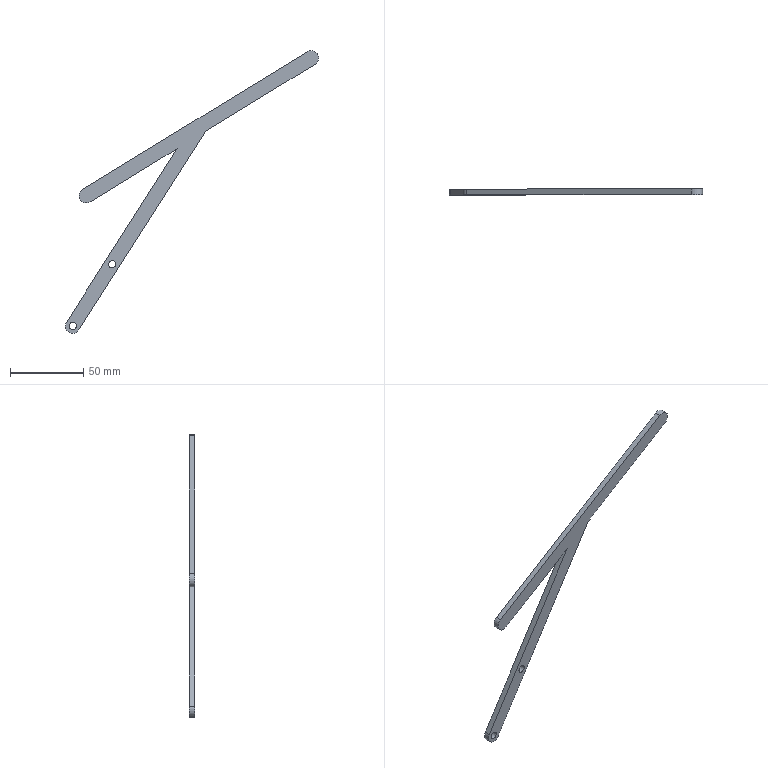Component | NX | WIPER | 1 solid | 12 faces | box 172.82 x 4 x 192.92 mm | volume 13538 mm3 | plane 7 | cylinder 5 | commonest cylinder face diameters 10 x3 5 x2
STEP:
#1=CARTESIAN_POINT('',(0.,0.,0.));
#2=DIRECTION('',(0.,0.,1.));
#3=DIRECTION('',(1.,0.,0.));
#4=AXIS2_PLACEMENT_3D('',#1,#2,#3);
#5=CARTESIAN_POINT('',(454.373,501.538,51.068));
#6=VERTEX_POINT('',#5);
#7=CARTESIAN_POINT('',(459.594,501.538,42.539));
#8=VERTEX_POINT('',#7);
#9=CARTESIAN_POINT('',(456.984,501.538,46.803));
#10=DIRECTION('',(0.,-1.,0.));
#11=DIRECTION('',(0.8431,0.,-0.5378));
#12=AXIS2_PLACEMENT_3D('',#9,#10,#11);
#13=CIRCLE('',#12,5.);
#14=CARTESIAN_POINT('',(456.984,497.538,46.803));
#15=DIRECTION('',(0.,1.,0.));
#16=DIRECTION('',(0.5378,0.,0.8431));
#17=AXIS2_PLACEMENT_3D('',#14,#15,#16);
#18=CYLINDRICAL_SURFACE('',#17,5.);
#19=CARTESIAN_POINT('',(7.854,4.));
#20=DIRECTION('',(-1.,0.));
#21=VECTOR('',#20,1.);
#22=LINE('',#19,#21);
#23=(GEOMETRIC_REPRESENTATION_CONTEXT(2)PARAMETRIC_REPRESENTATION_CONTEXT()REPRESENTATION_CONTEXT('',''));
#24=DEFINITIONAL_REPRESENTATION('',(#22),#23);
#25=PCURVE('',#18,#24);
#26=CARTESIAN_POINT('',(456.984,501.538,46.803));
#27=DIRECTION('',(0.,-1.,0.));
#28=DIRECTION('',(-0.5378,0.,-0.8431));
#29=AXIS2_PLACEMENT_3D('',#26,#27,#28);
#30=PLANE('',#29);
#31=CARTESIAN_POINT('',(0.,0.));
#32=DIRECTION('',(0.,1.));
#33=AXIS2_PLACEMENT_2D('',#31,#32);
#34=CIRCLE('',#33,5.);
#35=(GEOMETRIC_REPRESENTATION_CONTEXT(2)PARAMETRIC_REPRESENTATION_CONTEXT()REPRESENTATION_CONTEXT('',''));
#36=DEFINITIONAL_REPRESENTATION('',(#34),#35);
#37=PCURVE('',#30,#36);
#38=SURFACE_CURVE('',#13,(#25,#37),.PCURVE_S1.);
#39=EDGE_CURVE('',#6,#8,#38,.T.);
#40=ORIENTED_EDGE('',*,*,#39,.T.);
#41=CARTESIAN_POINT('',(459.594,497.538,42.539));
#42=VERTEX_POINT('',#41);
#43=CARTESIAN_POINT('',(459.594,497.538,42.539));
#44=DIRECTION('',(0.,1.,0.));
#45=VECTOR('',#44,1.);
#46=LINE('',#43,#45);
#47=CARTESIAN_POINT('',(2.025,0.));
#48=DIRECTION('',(0.,1.));
#49=VECTOR('',#48,1.);
#50=LINE('',#47,#49);
#51=(GEOMETRIC_REPRESENTATION_CONTEXT(2)PARAMETRIC_REPRESENTATION_CONTEXT()REPRESENTATION_CONTEXT('',''));
#52=DEFINITIONAL_REPRESENTATION('',(#50),#51);
#53=PCURVE('',#18,#52);
#54=CARTESIAN_POINT('',(459.594,497.538,42.539));
#55=DIRECTION('',(-0.522,0.,0.8529));
#56=DIRECTION('',(-0.8529,0.,-0.522));
#57=AXIS2_PLACEMENT_3D('',#54,#55,#56);
#58=PLANE('',#57);
#59=CARTESIAN_POINT('',(0.,0.));
#60=DIRECTION('',(0.,-1.));
#61=VECTOR('',#60,1.);
#62=LINE('',#59,#61);
#63=(GEOMETRIC_REPRESENTATION_CONTEXT(2)PARAMETRIC_REPRESENTATION_CONTEXT()REPRESENTATION_CONTEXT('',''));
#64=DEFINITIONAL_REPRESENTATION('',(#62),#63);
#65=PCURVE('',#58,#64);
#66=SURFACE_CURVE('',#46,(#53,#65),.PCURVE_S1.);
#67=EDGE_CURVE('',#42,#8,#66,.T.);
#68=ORIENTED_EDGE('',*,*,#67,.F.);
#69=CARTESIAN_POINT('',(454.373,497.538,51.068));
#70=VERTEX_POINT('',#69);
#71=CARTESIAN_POINT('',(456.984,497.538,46.803));
#72=DIRECTION('',(0.,-1.,0.));
#73=DIRECTION('',(0.8431,0.,-0.5378));
#74=AXIS2_PLACEMENT_3D('',#71,#72,#73);
#75=CIRCLE('',#74,5.);
#76=CARTESIAN_POINT('',(7.854,0.));
#77=DIRECTION('',(-1.,0.));
#78=VECTOR('',#77,1.);
#79=LINE('',#76,#78);
#80=(GEOMETRIC_REPRESENTATION_CONTEXT(2)PARAMETRIC_REPRESENTATION_CONTEXT()REPRESENTATION_CONTEXT('',''));
#81=DEFINITIONAL_REPRESENTATION('',(#79),#80);
#82=PCURVE('',#18,#81);
#83=CARTESIAN_POINT('',(456.984,497.538,46.803));
#84=DIRECTION('',(0.,-1.,0.));
#85=DIRECTION('',(-0.5378,0.,-0.8431));
#86=AXIS2_PLACEMENT_3D('',#83,#84,#85);
#87=PLANE('',#86);
#88=CARTESIAN_POINT('',(0.,0.));
#89=DIRECTION('',(0.,1.));
#90=AXIS2_PLACEMENT_2D('',#88,#89);
#91=CIRCLE('',#90,5.);
#92=(GEOMETRIC_REPRESENTATION_CONTEXT(2)PARAMETRIC_REPRESENTATION_CONTEXT()REPRESENTATION_CONTEXT('',''));
#93=DEFINITIONAL_REPRESENTATION('',(#91),#92);
#94=PCURVE('',#87,#93);
#95=SURFACE_CURVE('',#75,(#82,#94),.PCURVE_S1.);
#96=EDGE_CURVE('',#70,#42,#95,.T.);
#97=ORIENTED_EDGE('',*,*,#96,.F.);
#98=CARTESIAN_POINT('',(454.373,497.538,51.068));
#99=DIRECTION('',(0.,1.,0.));
#100=VECTOR('',#99,1.);
#101=LINE('',#98,#100);
#102=CARTESIAN_POINT('',(5.166,0.));
#103=DIRECTION('',(0.,1.));
#104=VECTOR('',#103,1.);
#105=LINE('',#102,#104);
#106=(GEOMETRIC_REPRESENTATION_CONTEXT(2)PARAMETRIC_REPRESENTATION_CONTEXT()REPRESENTATION_CONTEXT('',''));
#107=DEFINITIONAL_REPRESENTATION('',(#105),#106);
#108=PCURVE('',#18,#107);
#109=CARTESIAN_POINT('',(607.901,497.538,145.033));
#110=DIRECTION('',(0.522,0.,-0.8529));
#111=DIRECTION('',(0.8529,0.,0.522));
#112=AXIS2_PLACEMENT_3D('',#109,#110,#111);
#113=PLANE('',#112);
#114=CARTESIAN_POINT('',(-180.,0.));
#115=DIRECTION('',(0.,-1.));
#116=VECTOR('',#115,1.);
#117=LINE('',#114,#116);
#118=(GEOMETRIC_REPRESENTATION_CONTEXT(2)PARAMETRIC_REPRESENTATION_CONTEXT()REPRESENTATION_CONTEXT('',''));
#119=DEFINITIONAL_REPRESENTATION('',(#117),#118);
#120=PCURVE('',#113,#119);
#121=SURFACE_CURVE('',#101,(#108,#120),.PCURVE_S1.);
#122=EDGE_CURVE('',#70,#6,#121,.T.);
#123=ORIENTED_EDGE('',*,*,#122,.T.);
#124=EDGE_LOOP('',(#40,#68,#97,#123));
#125=FACE_BOUND('',#124,.T.);
#126=ADVANCED_FACE('',(#125),#18,.T.);
#127=CARTESIAN_POINT('',(518.949,501.538,78.866));
#128=VERTEX_POINT('',#127);
#129=CARTESIAN_POINT('',(459.594,501.538,42.539));
#130=DIRECTION('',(0.8529,0.,0.522));
#131=VECTOR('',#130,1.);
#132=LINE('',#129,#131);
#133=CARTESIAN_POINT('',(0.,-4.));
#134=DIRECTION('',(-1.,0.));
#135=VECTOR('',#134,1.);
#136=LINE('',#133,#135);
#137=(GEOMETRIC_REPRESENTATION_CONTEXT(2)PARAMETRIC_REPRESENTATION_CONTEXT()REPRESENTATION_CONTEXT('',''));
#138=DEFINITIONAL_REPRESENTATION('',(#136),#137);
#139=PCURVE('',#58,#138);
#140=CARTESIAN_POINT('',(2.192,4.494));
#141=DIRECTION('',(-0.8988,0.4384));
#142=VECTOR('',#141,1.);
#143=LINE('',#140,#142);
#144=(GEOMETRIC_REPRESENTATION_CONTEXT(2)PARAMETRIC_REPRESENTATION_CONTEXT()REPRESENTATION_CONTEXT('',''));
#145=DEFINITIONAL_REPRESENTATION('',(#143),#144);
#146=PCURVE('',#30,#145);
#147=SURFACE_CURVE('',#132,(#139,#146),.PCURVE_S1.);
#148=EDGE_CURVE('',#8,#128,#147,.T.);
#149=ORIENTED_EDGE('',*,*,#148,.T.);
#150=CARTESIAN_POINT('',(518.949,497.538,78.866));
#151=VERTEX_POINT('',#150);
#152=CARTESIAN_POINT('',(518.949,497.538,78.866));
#153=DIRECTION('',(0.,1.,0.));
#154=VECTOR('',#153,1.);
#155=LINE('',#152,#154);
#156=CARTESIAN_POINT('',(-69.59,0.));
#157=DIRECTION('',(0.,-1.));
#158=VECTOR('',#157,1.);
#159=LINE('',#156,#158);
#160=(GEOMETRIC_REPRESENTATION_CONTEXT(2)PARAMETRIC_REPRESENTATION_CONTEXT()REPRESENTATION_CONTEXT('',''));
#161=DEFINITIONAL_REPRESENTATION('',(#159),#160);
#162=PCURVE('',#58,#161);
#163=CARTESIAN_POINT('',(518.949,497.538,78.866));
#164=DIRECTION('',(0.8431,0.,-0.5378));
#165=DIRECTION('',(0.5378,0.,0.8431));
#166=AXIS2_PLACEMENT_3D('',#163,#164,#165);
#167=PLANE('',#166);
#168=CARTESIAN_POINT('',(0.,0.));
#169=DIRECTION('',(0.,-1.));
#170=VECTOR('',#169,1.);
#171=LINE('',#168,#170);
#172=(GEOMETRIC_REPRESENTATION_CONTEXT(2)PARAMETRIC_REPRESENTATION_CONTEXT()REPRESENTATION_CONTEXT('',''));
#173=DEFINITIONAL_REPRESENTATION('',(#171),#172);
#174=PCURVE('',#167,#173);
#175=SURFACE_CURVE('',#155,(#162,#174),.PCURVE_S1.);
#176=EDGE_CURVE('',#151,#128,#175,.T.);
#177=ORIENTED_EDGE('',*,*,#176,.F.);
#178=CARTESIAN_POINT('',(459.594,497.538,42.539));
#179=DIRECTION('',(0.8529,0.,0.522));
#180=VECTOR('',#179,1.);
#181=LINE('',#178,#180);
#182=CARTESIAN_POINT('',(0.,0.));
#183=DIRECTION('',(-1.,0.));
#184=VECTOR('',#183,1.);
#185=LINE('',#182,#184);
#186=(GEOMETRIC_REPRESENTATION_CONTEXT(2)PARAMETRIC_REPRESENTATION_CONTEXT()REPRESENTATION_CONTEXT('',''));
#187=DEFINITIONAL_REPRESENTATION('',(#185),#186);
#188=PCURVE('',#58,#187);
#189=CARTESIAN_POINT('',(2.192,4.494));
#190=DIRECTION('',(-0.8988,0.4384));
#191=VECTOR('',#190,1.);
#192=LINE('',#189,#191);
#193=(GEOMETRIC_REPRESENTATION_CONTEXT(2)PARAMETRIC_REPRESENTATION_CONTEXT()REPRESENTATION_CONTEXT('',''));
#194=DEFINITIONAL_REPRESENTATION('',(#192),#193);
#195=PCURVE('',#87,#194);
#196=SURFACE_CURVE('',#181,(#188,#195),.PCURVE_S1.);
#197=EDGE_CURVE('',#42,#151,#196,.T.);
#198=ORIENTED_EDGE('',*,*,#197,.F.);
#199=ORIENTED_EDGE('',*,*,#67,.T.);
#200=EDGE_LOOP('',(#149,#177,#198,#199));
#201=FACE_BOUND('',#200,.T.);
#202=ADVANCED_FACE('',(#201),#58,.F.);
#203=CARTESIAN_POINT('',(443.471,501.538,-39.466));
#204=VERTEX_POINT('',#203);
#205=CARTESIAN_POINT('',(518.949,501.538,78.866));
#206=DIRECTION('',(-0.5378,0.,-0.8431));
#207=VECTOR('',#206,1.);
#208=LINE('',#205,#207);
#209=CARTESIAN_POINT('',(0.,-4.));
#210=DIRECTION('',(-1.,0.));
#211=VECTOR('',#210,1.);
#212=LINE('',#209,#211);
#213=(GEOMETRIC_REPRESENTATION_CONTEXT(2)PARAMETRIC_REPRESENTATION_CONTEXT()REPRESENTATION_CONTEXT('',''));
#214=DEFINITIONAL_REPRESENTATION('',(#212),#213);
#215=PCURVE('',#167,#214);
#216=CARTESIAN_POINT('',(-60.355,35.));
#217=DIRECTION('',(1.,0.));
#218=VECTOR('',#217,1.);
#219=LINE('',#216,#218);
#220=(GEOMETRIC_REPRESENTATION_CONTEXT(2)PARAMETRIC_REPRESENTATION_CONTEXT()REPRESENTATION_CONTEXT('',''));
#221=DEFINITIONAL_REPRESENTATION('',(#219),#220);
#222=PCURVE('',#30,#221);
#223=SURFACE_CURVE('',#208,(#215,#222),.PCURVE_S1.);
#224=EDGE_CURVE('',#128,#204,#223,.T.);
#225=ORIENTED_EDGE('',*,*,#224,.T.);
#226=CARTESIAN_POINT('',(443.471,497.538,-39.466));
#227=VERTEX_POINT('',#226);
#228=CARTESIAN_POINT('',(443.471,497.538,-39.466));
#229=DIRECTION('',(0.,1.,0.));
#230=VECTOR('',#229,1.);
#231=LINE('',#228,#230);
#232=CARTESIAN_POINT('',(-140.355,0.));
#233=DIRECTION('',(0.,-1.));
#234=VECTOR('',#233,1.);
#235=LINE('',#232,#234);
#236=(GEOMETRIC_REPRESENTATION_CONTEXT(2)PARAMETRIC_REPRESENTATION_CONTEXT()REPRESENTATION_CONTEXT('',''));
#237=DEFINITIONAL_REPRESENTATION('',(#235),#236);
#238=PCURVE('',#167,#237);
#239=CARTESIAN_POINT('',(447.686,497.538,-42.155));
#240=DIRECTION('',(0.,1.,0.));
#241=DIRECTION('',(0.5378,0.,0.8431));
#242=AXIS2_PLACEMENT_3D('',#239,#240,#241);
#243=CYLINDRICAL_SURFACE('',#242,5.);
#244=CARTESIAN_POINT('',(4.712,0.));
#245=DIRECTION('',(0.,1.));
#246=VECTOR('',#245,1.);
#247=LINE('',#244,#246);
#248=(GEOMETRIC_REPRESENTATION_CONTEXT(2)PARAMETRIC_REPRESENTATION_CONTEXT()REPRESENTATION_CONTEXT('',''));
#249=DEFINITIONAL_REPRESENTATION('',(#247),#248);
#250=PCURVE('',#243,#249);
#251=SURFACE_CURVE('',#231,(#238,#250),.PCURVE_S1.);
#252=EDGE_CURVE('',#227,#204,#251,.T.);
#253=ORIENTED_EDGE('',*,*,#252,.F.);
#254=CARTESIAN_POINT('',(518.949,497.538,78.866));
#255=DIRECTION('',(-0.5378,0.,-0.8431));
#256=VECTOR('',#255,1.);
#257=LINE('',#254,#256);
#258=CARTESIAN_POINT('',(0.,0.));
#259=DIRECTION('',(-1.,0.));
#260=VECTOR('',#259,1.);
#261=LINE('',#258,#260);
#262=(GEOMETRIC_REPRESENTATION_CONTEXT(2)PARAMETRIC_REPRESENTATION_CONTEXT()REPRESENTATION_CONTEXT('',''));
#263=DEFINITIONAL_REPRESENTATION('',(#261),#262);
#264=PCURVE('',#167,#263);
#265=CARTESIAN_POINT('',(-60.355,35.));
#266=DIRECTION('',(1.,0.));
#267=VECTOR('',#266,1.);
#268=LINE('',#265,#267);
#269=(GEOMETRIC_REPRESENTATION_CONTEXT(2)PARAMETRIC_REPRESENTATION_CONTEXT()REPRESENTATION_CONTEXT('',''));
#270=DEFINITIONAL_REPRESENTATION('',(#268),#269);
#271=PCURVE('',#87,#270);
#272=SURFACE_CURVE('',#257,(#264,#271),.PCURVE_S1.);
#273=EDGE_CURVE('',#151,#227,#272,.T.);
#274=ORIENTED_EDGE('',*,*,#273,.F.);
#275=ORIENTED_EDGE('',*,*,#176,.T.);
#276=EDGE_LOOP('',(#225,#253,#274,#275));
#277=FACE_BOUND('',#276,.T.);
#278=ADVANCED_FACE('',(#277),#167,.F.);
#279=CARTESIAN_POINT('',(451.901,501.538,-44.844));
#280=VERTEX_POINT('',#279);
#281=CARTESIAN_POINT('',(447.686,501.538,-42.155));
#282=DIRECTION('',(0.,-1.,0.));
#283=DIRECTION('',(0.8431,0.,-0.5378));
#284=AXIS2_PLACEMENT_3D('',#281,#282,#283);
#285=CIRCLE('',#284,5.);
#286=CARTESIAN_POINT('',(7.854,4.));
#287=DIRECTION('',(-1.,0.));
#288=VECTOR('',#287,1.);
#289=LINE('',#286,#288);
#290=(GEOMETRIC_REPRESENTATION_CONTEXT(2)PARAMETRIC_REPRESENTATION_CONTEXT()REPRESENTATION_CONTEXT('',''));
#291=DEFINITIONAL_REPRESENTATION('',(#289),#290);
#292=PCURVE('',#243,#291);
#293=CARTESIAN_POINT('',(80.,40.));
#294=DIRECTION('',(0.,1.));
#295=AXIS2_PLACEMENT_2D('',#293,#294);
#296=CIRCLE('',#295,5.);
#297=(GEOMETRIC_REPRESENTATION_CONTEXT(2)PARAMETRIC_REPRESENTATION_CONTEXT()REPRESENTATION_CONTEXT('',''));
#298=DEFINITIONAL_REPRESENTATION('',(#296),#297);
#299=PCURVE('',#30,#298);
#300=SURFACE_CURVE('',#285,(#292,#299),.PCURVE_S1.);
#301=EDGE_CURVE('',#204,#280,#300,.T.);
#302=ORIENTED_EDGE('',*,*,#301,.T.);
#303=CARTESIAN_POINT('',(451.901,497.538,-44.844));
#304=VERTEX_POINT('',#303);
#305=CARTESIAN_POINT('',(451.901,497.538,-44.844));
#306=DIRECTION('',(0.,1.,0.));
#307=VECTOR('',#306,1.);
#308=LINE('',#305,#307);
#309=CARTESIAN_POINT('',(1.571,0.));
#310=DIRECTION('',(0.,1.));
#311=VECTOR('',#310,1.);
#312=LINE('',#309,#311);
#313=(GEOMETRIC_REPRESENTATION_CONTEXT(2)PARAMETRIC_REPRESENTATION_CONTEXT()REPRESENTATION_CONTEXT('',''));
#314=DEFINITIONAL_REPRESENTATION('',(#312),#313);
#315=PCURVE('',#243,#314);
#316=CARTESIAN_POINT('',(451.901,497.538,-44.844));
#317=DIRECTION('',(-0.8431,0.,0.5378));
#318=DIRECTION('',(-0.5378,0.,-0.8431));
#319=AXIS2_PLACEMENT_3D('',#316,#317,#318);
#320=PLANE('',#319);
#321=CARTESIAN_POINT('',(0.,0.));
#322=DIRECTION('',(0.,-1.));
#323=VECTOR('',#322,1.);
#324=LINE('',#321,#323);
#325=(GEOMETRIC_REPRESENTATION_CONTEXT(2)PARAMETRIC_REPRESENTATION_CONTEXT()REPRESENTATION_CONTEXT('',''));
#326=DEFINITIONAL_REPRESENTATION('',(#324),#325);
#327=PCURVE('',#320,#326);
#328=SURFACE_CURVE('',#308,(#315,#327),.PCURVE_S1.);
#329=EDGE_CURVE('',#304,#280,#328,.T.);
#330=ORIENTED_EDGE('',*,*,#329,.F.);
#331=CARTESIAN_POINT('',(447.686,497.538,-42.155));
#332=DIRECTION('',(0.,-1.,0.));
#333=DIRECTION('',(0.8431,0.,-0.5378));
#334=AXIS2_PLACEMENT_3D('',#331,#332,#333);
#335=CIRCLE('',#334,5.);
#336=CARTESIAN_POINT('',(7.854,0.));
#337=DIRECTION('',(-1.,0.));
#338=VECTOR('',#337,1.);
#339=LINE('',#336,#338);
#340=(GEOMETRIC_REPRESENTATION_CONTEXT(2)PARAMETRIC_REPRESENTATION_CONTEXT()REPRESENTATION_CONTEXT('',''));
#341=DEFINITIONAL_REPRESENTATION('',(#339),#340);
#342=PCURVE('',#243,#341);
#343=CARTESIAN_POINT('',(80.,40.));
#344=DIRECTION('',(0.,1.));
#345=AXIS2_PLACEMENT_2D('',#343,#344);
#346=CIRCLE('',#345,5.);
#347=(GEOMETRIC_REPRESENTATION_CONTEXT(2)PARAMETRIC_REPRESENTATION_CONTEXT()REPRESENTATION_CONTEXT('',''));
#348=DEFINITIONAL_REPRESENTATION('',(#346),#347);
#349=PCURVE('',#87,#348);
#350=SURFACE_CURVE('',#335,(#342,#349),.PCURVE_S1.);
#351=EDGE_CURVE('',#227,#304,#350,.T.);
#352=ORIENTED_EDGE('',*,*,#351,.F.);
#353=ORIENTED_EDGE('',*,*,#252,.T.);
#354=EDGE_LOOP('',(#302,#330,#352,#353));
#355=FACE_BOUND('',#354,.T.);
#356=ADVANCED_FACE('',(#355),#243,.T.);
#357=CARTESIAN_POINT('',(538.405,501.538,90.775));
#358=VERTEX_POINT('',#357);
#359=CARTESIAN_POINT('',(451.901,501.538,-44.844));
#360=DIRECTION('',(0.5378,0.,0.8431));
#361=VECTOR('',#360,1.);
#362=LINE('',#359,#361);
#363=CARTESIAN_POINT('',(0.,-4.));
#364=DIRECTION('',(-1.,0.));
#365=VECTOR('',#364,1.);
#366=LINE('',#363,#365);
#367=(GEOMETRIC_REPRESENTATION_CONTEXT(2)PARAMETRIC_REPRESENTATION_CONTEXT()REPRESENTATION_CONTEXT('',''));
#368=DEFINITIONAL_REPRESENTATION('',(#366),#367);
#369=PCURVE('',#320,#368);
#370=CARTESIAN_POINT('',(80.,45.));
#371=DIRECTION('',(-1.,0.));
#372=VECTOR('',#371,1.);
#373=LINE('',#370,#372);
#374=(GEOMETRIC_REPRESENTATION_CONTEXT(2)PARAMETRIC_REPRESENTATION_CONTEXT()REPRESENTATION_CONTEXT('',''));
#375=DEFINITIONAL_REPRESENTATION('',(#373),#374);
#376=PCURVE('',#30,#375);
#377=SURFACE_CURVE('',#362,(#369,#376),.PCURVE_S1.);
#378=EDGE_CURVE('',#280,#358,#377,.T.);
#379=ORIENTED_EDGE('',*,*,#378,.T.);
#380=CARTESIAN_POINT('',(538.405,497.538,90.775));
#381=VERTEX_POINT('',#380);
#382=CARTESIAN_POINT('',(538.405,497.538,90.775));
#383=DIRECTION('',(0.,1.,0.));
#384=VECTOR('',#383,1.);
#385=LINE('',#382,#384);
#386=CARTESIAN_POINT('',(-160.858,0.));
#387=DIRECTION('',(0.,-1.));
#388=VECTOR('',#387,1.);
#389=LINE('',#386,#388);
#390=(GEOMETRIC_REPRESENTATION_CONTEXT(2)PARAMETRIC_REPRESENTATION_CONTEXT()REPRESENTATION_CONTEXT('',''));
#391=DEFINITIONAL_REPRESENTATION('',(#389),#390);
#392=PCURVE('',#320,#391);
#393=CARTESIAN_POINT('',(538.405,497.538,90.775));
#394=DIRECTION('',(-0.522,0.,0.8529));
#395=DIRECTION('',(-0.8529,0.,-0.522));
#396=AXIS2_PLACEMENT_3D('',#393,#394,#395);
#397=PLANE('',#396);
#398=CARTESIAN_POINT('',(0.,0.));
#399=DIRECTION('',(0.,-1.));
#400=VECTOR('',#399,1.);
#401=LINE('',#398,#400);
#402=(GEOMETRIC_REPRESENTATION_CONTEXT(2)PARAMETRIC_REPRESENTATION_CONTEXT()REPRESENTATION_CONTEXT('',''));
#403=DEFINITIONAL_REPRESENTATION('',(#401),#402);
#404=PCURVE('',#397,#403);
#405=SURFACE_CURVE('',#385,(#392,#404),.PCURVE_S1.);
#406=EDGE_CURVE('',#381,#358,#405,.T.);
#407=ORIENTED_EDGE('',*,*,#406,.F.);
#408=CARTESIAN_POINT('',(451.901,497.538,-44.844));
#409=DIRECTION('',(0.5378,0.,0.8431));
#410=VECTOR('',#409,1.);
#411=LINE('',#408,#410);
#412=CARTESIAN_POINT('',(0.,0.));
#413=DIRECTION('',(-1.,0.));
#414=VECTOR('',#413,1.);
#415=LINE('',#412,#414);
#416=(GEOMETRIC_REPRESENTATION_CONTEXT(2)PARAMETRIC_REPRESENTATION_CONTEXT()REPRESENTATION_CONTEXT('',''));
#417=DEFINITIONAL_REPRESENTATION('',(#415),#416);
#418=PCURVE('',#320,#417);
#419=CARTESIAN_POINT('',(80.,45.));
#420=DIRECTION('',(-1.,0.));
#421=VECTOR('',#420,1.);
#422=LINE('',#419,#421);
#423=(GEOMETRIC_REPRESENTATION_CONTEXT(2)PARAMETRIC_REPRESENTATION_CONTEXT()REPRESENTATION_CONTEXT('',''));
#424=DEFINITIONAL_REPRESENTATION('',(#422),#423);
#425=PCURVE('',#87,#424);
#426=SURFACE_CURVE('',#411,(#418,#425),.PCURVE_S1.);
#427=EDGE_CURVE('',#304,#381,#426,.T.);
#428=ORIENTED_EDGE('',*,*,#427,.F.);
#429=ORIENTED_EDGE('',*,*,#329,.T.);
#430=EDGE_LOOP('',(#379,#407,#428,#429));
#431=FACE_BOUND('',#430,.T.);
#432=ADVANCED_FACE('',(#431),#320,.F.);
#433=CARTESIAN_POINT('',(613.121,501.538,136.504));
#434=VERTEX_POINT('',#433);
#435=CARTESIAN_POINT('',(538.405,501.538,90.775));
#436=DIRECTION('',(0.8529,0.,0.522));
#437=VECTOR('',#436,1.);
#438=LINE('',#435,#437);
#439=CARTESIAN_POINT('',(0.,-4.));
#440=DIRECTION('',(-1.,0.));
#441=VECTOR('',#440,1.);
#442=LINE('',#439,#441);
#443=(GEOMETRIC_REPRESENTATION_CONTEXT(2)PARAMETRIC_REPRESENTATION_CONTEXT()REPRESENTATION_CONTEXT('',''));
#444=DEFINITIONAL_REPRESENTATION('',(#442),#443);
#445=PCURVE('',#397,#444);
#446=CARTESIAN_POINT('',(-80.858,45.));
#447=DIRECTION('',(-0.8988,0.4384));
#448=VECTOR('',#447,1.);
#449=LINE('',#446,#448);
#450=(GEOMETRIC_REPRESENTATION_CONTEXT(2)PARAMETRIC_REPRESENTATION_CONTEXT()REPRESENTATION_CONTEXT('',''));
#451=DEFINITIONAL_REPRESENTATION('',(#449),#450);
#452=PCURVE('',#30,#451);
#453=SURFACE_CURVE('',#438,(#445,#452),.PCURVE_S1.);
#454=EDGE_CURVE('',#358,#434,#453,.T.);
#455=ORIENTED_EDGE('',*,*,#454,.T.);
#456=CARTESIAN_POINT('',(613.121,497.538,136.504));
#457=VERTEX_POINT('',#456);
#458=CARTESIAN_POINT('',(613.121,497.538,136.504));
#459=DIRECTION('',(0.,1.,0.));
#460=VECTOR('',#459,1.);
#461=LINE('',#458,#460);
#462=CARTESIAN_POINT('',(-87.599,0.));
#463=DIRECTION('',(0.,-1.));
#464=VECTOR('',#463,1.);
#465=LINE('',#462,#464);
#466=(GEOMETRIC_REPRESENTATION_CONTEXT(2)PARAMETRIC_REPRESENTATION_CONTEXT()REPRESENTATION_CONTEXT('',''));
#467=DEFINITIONAL_REPRESENTATION('',(#465),#466);
#468=PCURVE('',#397,#467);
#469=CARTESIAN_POINT('',(610.511,497.538,140.768));
#470=DIRECTION('',(0.,1.,0.));
#471=DIRECTION('',(0.5378,0.,0.8431));
#472=AXIS2_PLACEMENT_3D('',#469,#470,#471);
#473=CYLINDRICAL_SURFACE('',#472,5.);
#474=CARTESIAN_POINT('',(2.025,0.));
#475=DIRECTION('',(0.,1.));
#476=VECTOR('',#475,1.);
#477=LINE('',#474,#476);
#478=(GEOMETRIC_REPRESENTATION_CONTEXT(2)PARAMETRIC_REPRESENTATION_CONTEXT()REPRESENTATION_CONTEXT('',''));
#479=DEFINITIONAL_REPRESENTATION('',(#477),#478);
#480=PCURVE('',#473,#479);
#481=SURFACE_CURVE('',#461,(#468,#480),.PCURVE_S1.);
#482=EDGE_CURVE('',#457,#434,#481,.T.);
#483=ORIENTED_EDGE('',*,*,#482,.F.);
#484=CARTESIAN_POINT('',(538.405,497.538,90.775));
#485=DIRECTION('',(0.8529,0.,0.522));
#486=VECTOR('',#485,1.);
#487=LINE('',#484,#486);
#488=CARTESIAN_POINT('',(0.,0.));
#489=DIRECTION('',(-1.,0.));
#490=VECTOR('',#489,1.);
#491=LINE('',#488,#490);
#492=(GEOMETRIC_REPRESENTATION_CONTEXT(2)PARAMETRIC_REPRESENTATION_CONTEXT()REPRESENTATION_CONTEXT('',''));
#493=DEFINITIONAL_REPRESENTATION('',(#491),#492);
#494=PCURVE('',#397,#493);
#495=CARTESIAN_POINT('',(-80.858,45.));
#496=DIRECTION('',(-0.8988,0.4384));
#497=VECTOR('',#496,1.);
#498=LINE('',#495,#497);
#499=(GEOMETRIC_REPRESENTATION_CONTEXT(2)PARAMETRIC_REPRESENTATION_CONTEXT()REPRESENTATION_CONTEXT('',''));
#500=DEFINITIONAL_REPRESENTATION('',(#498),#499);
#501=PCURVE('',#87,#500);
#502=SURFACE_CURVE('',#487,(#494,#501),.PCURVE_S1.);
#503=EDGE_CURVE('',#381,#457,#502,.T.);
#504=ORIENTED_EDGE('',*,*,#503,.F.);
#505=ORIENTED_EDGE('',*,*,#406,.T.);
#506=EDGE_LOOP('',(#455,#483,#504,#505));
#507=FACE_BOUND('',#506,.T.);
#508=ADVANCED_FACE('',(#507),#397,.F.);
#509=CARTESIAN_POINT('',(607.901,501.538,145.033));
#510=VERTEX_POINT('',#509);
#511=CARTESIAN_POINT('',(610.511,501.538,140.768));
#512=DIRECTION('',(0.,-1.,0.));
#513=DIRECTION('',(0.8431,0.,-0.5378));
#514=AXIS2_PLACEMENT_3D('',#511,#512,#513);
#515=CIRCLE('',#514,5.);
#516=CARTESIAN_POINT('',(7.854,4.));
#517=DIRECTION('',(-1.,0.));
#518=VECTOR('',#517,1.);
#519=LINE('',#516,#518);
#520=(GEOMETRIC_REPRESENTATION_CONTEXT(2)PARAMETRIC_REPRESENTATION_CONTEXT()REPRESENTATION_CONTEXT('',''));
#521=DEFINITIONAL_REPRESENTATION('',(#519),#520);
#522=PCURVE('',#473,#521);
#523=CARTESIAN_POINT('',(-161.783,78.907));
#524=DIRECTION('',(-0.,1.));
#525=AXIS2_PLACEMENT_2D('',#523,#524);
#526=CIRCLE('',#525,5.);
#527=(GEOMETRIC_REPRESENTATION_CONTEXT(2)PARAMETRIC_REPRESENTATION_CONTEXT()REPRESENTATION_CONTEXT('',''));
#528=DEFINITIONAL_REPRESENTATION('',(#526),#527);
#529=PCURVE('',#30,#528);
#530=SURFACE_CURVE('',#515,(#522,#529),.PCURVE_S1.);
#531=EDGE_CURVE('',#434,#510,#530,.T.);
#532=ORIENTED_EDGE('',*,*,#531,.T.);
#533=CARTESIAN_POINT('',(607.901,497.538,145.033));
#534=VERTEX_POINT('',#533);
#535=CARTESIAN_POINT('',(607.901,497.538,145.033));
#536=DIRECTION('',(0.,1.,0.));
#537=VECTOR('',#536,1.);
#538=LINE('',#535,#537);
#539=CARTESIAN_POINT('',(-1.117,0.));
#540=DIRECTION('',(0.,1.));
#541=VECTOR('',#540,1.);
#542=LINE('',#539,#541);
#543=(GEOMETRIC_REPRESENTATION_CONTEXT(2)PARAMETRIC_REPRESENTATION_CONTEXT()REPRESENTATION_CONTEXT('',''));
#544=DEFINITIONAL_REPRESENTATION('',(#542),#543);
#545=PCURVE('',#473,#544);
#546=CARTESIAN_POINT('',(0.,0.));
#547=DIRECTION('',(0.,-1.));
#548=VECTOR('',#547,1.);
#549=LINE('',#546,#548);
#550=(GEOMETRIC_REPRESENTATION_CONTEXT(2)PARAMETRIC_REPRESENTATION_CONTEXT()REPRESENTATION_CONTEXT('',''));
#551=DEFINITIONAL_REPRESENTATION('',(#549),#550);
#552=PCURVE('',#113,#551);
#553=SURFACE_CURVE('',#538,(#545,#552),.PCURVE_S1.);
#554=EDGE_CURVE('',#534,#510,#553,.T.);
#555=ORIENTED_EDGE('',*,*,#554,.F.);
#556=CARTESIAN_POINT('',(610.511,497.538,140.768));
#557=DIRECTION('',(0.,-1.,0.));
#558=DIRECTION('',(0.8431,0.,-0.5378));
#559=AXIS2_PLACEMENT_3D('',#556,#557,#558);
#560=CIRCLE('',#559,5.);
#561=CARTESIAN_POINT('',(7.854,0.));
#562=DIRECTION('',(-1.,0.));
#563=VECTOR('',#562,1.);
#564=LINE('',#561,#563);
#565=(GEOMETRIC_REPRESENTATION_CONTEXT(2)PARAMETRIC_REPRESENTATION_CONTEXT()REPRESENTATION_CONTEXT('',''));
#566=DEFINITIONAL_REPRESENTATION('',(#564),#565);
#567=PCURVE('',#473,#566);
#568=CARTESIAN_POINT('',(-161.783,78.907));
#569=DIRECTION('',(-0.,1.));
#570=AXIS2_PLACEMENT_2D('',#568,#569);
#571=CIRCLE('',#570,5.);
#572=(GEOMETRIC_REPRESENTATION_CONTEXT(2)PARAMETRIC_REPRESENTATION_CONTEXT()REPRESENTATION_CONTEXT('',''));
#573=DEFINITIONAL_REPRESENTATION('',(#571),#572);
#574=PCURVE('',#87,#573);
#575=SURFACE_CURVE('',#560,(#567,#574),.PCURVE_S1.);
#576=EDGE_CURVE('',#457,#534,#575,.T.);
#577=ORIENTED_EDGE('',*,*,#576,.F.);
#578=ORIENTED_EDGE('',*,*,#482,.T.);
#579=EDGE_LOOP('',(#532,#555,#577,#578));
#580=FACE_BOUND('',#579,.T.);
#581=ADVANCED_FACE('',(#580),#473,.T.);
#582=CARTESIAN_POINT('',(449.794,497.538,-43.499));
#583=VERTEX_POINT('',#582);
#584=CARTESIAN_POINT('',(447.686,497.538,-42.155));
#585=DIRECTION('',(0.,-1.,0.));
#586=DIRECTION('',(0.8431,0.,-0.5378));
#587=AXIS2_PLACEMENT_3D('',#584,#585,#586);
#588=CIRCLE('',#587,2.5);
#589=CARTESIAN_POINT('',(447.686,497.538,-42.155));
#590=DIRECTION('',(0.,1.,0.));
#591=DIRECTION('',(0.5378,0.,0.8431));
#592=AXIS2_PLACEMENT_3D('',#589,#590,#591);
#593=CYLINDRICAL_SURFACE('',#592,2.5);
#594=CARTESIAN_POINT('',(7.854,0.));
#595=DIRECTION('',(-1.,0.));
#596=VECTOR('',#595,1.);
#597=LINE('',#594,#596);
#598=(GEOMETRIC_REPRESENTATION_CONTEXT(2)PARAMETRIC_REPRESENTATION_CONTEXT()REPRESENTATION_CONTEXT('',''));
#599=DEFINITIONAL_REPRESENTATION('',(#597),#598);
#600=PCURVE('',#593,#599);
#601=CARTESIAN_POINT('',(80.,40.));
#602=DIRECTION('',(0.,1.));
#603=AXIS2_PLACEMENT_2D('',#601,#602);
#604=CIRCLE('',#603,2.5);
#605=(GEOMETRIC_REPRESENTATION_CONTEXT(2)PARAMETRIC_REPRESENTATION_CONTEXT()REPRESENTATION_CONTEXT('',''));
#606=DEFINITIONAL_REPRESENTATION('',(#604),#605);
#607=PCURVE('',#87,#606);
#608=SURFACE_CURVE('',#588,(#600,#607),.PCURVE_S1.);
#609=EDGE_CURVE('',#583,#583,#608,.T.);
#610=ORIENTED_EDGE('',*,*,#609,.F.);
#611=CARTESIAN_POINT('',(449.794,501.538,-43.499));
#612=VERTEX_POINT('',#611);
#613=CARTESIAN_POINT('',(449.794,497.538,-43.499));
#614=CARTESIAN_POINT('',(449.794,501.538,-43.499));
#615=B_SPLINE_CURVE_WITH_KNOTS('',1,(#613,#614),.UNSPECIFIED.,.F.,.F.,(2,2),(0.,4.),.PIECEWISE_BEZIER_KNOTS.);
#616=CARTESIAN_POINT('',(7.854,0.));
#617=DIRECTION('',(0.,1.));
#618=VECTOR('',#617,1.);
#619=LINE('',#616,#618);
#620=(GEOMETRIC_REPRESENTATION_CONTEXT(2)PARAMETRIC_REPRESENTATION_CONTEXT()REPRESENTATION_CONTEXT('',''));
#621=DEFINITIONAL_REPRESENTATION('',(#619),#620);
#622=PCURVE('',#593,#621);
#623=CARTESIAN_POINT('',(1.571,0.));
#624=DIRECTION('',(0.,1.));
#625=VECTOR('',#624,1.);
#626=LINE('',#623,#625);
#627=(GEOMETRIC_REPRESENTATION_CONTEXT(2)PARAMETRIC_REPRESENTATION_CONTEXT()REPRESENTATION_CONTEXT('',''));
#628=DEFINITIONAL_REPRESENTATION('',(#626),#627);
#629=PCURVE('',#593,#628);
#630=SEAM_CURVE('',#615,(#622,#629),.PCURVE_S1.);
#631=EDGE_CURVE('',#583,#612,#630,.T.);
#632=ORIENTED_EDGE('',*,*,#631,.T.);
#633=CARTESIAN_POINT('',(447.686,501.538,-42.155));
#634=DIRECTION('',(0.,-1.,0.));
#635=DIRECTION('',(0.8431,0.,-0.5378));
#636=AXIS2_PLACEMENT_3D('',#633,#634,#635);
#637=CIRCLE('',#636,2.5);
#638=CARTESIAN_POINT('',(7.854,4.));
#639=DIRECTION('',(-1.,0.));
#640=VECTOR('',#639,1.);
#641=LINE('',#638,#640);
#642=(GEOMETRIC_REPRESENTATION_CONTEXT(2)PARAMETRIC_REPRESENTATION_CONTEXT()REPRESENTATION_CONTEXT('',''));
#643=DEFINITIONAL_REPRESENTATION('',(#641),#642);
#644=PCURVE('',#593,#643);
#645=CARTESIAN_POINT('',(80.,40.));
#646=DIRECTION('',(0.,1.));
#647=AXIS2_PLACEMENT_2D('',#645,#646);
#648=CIRCLE('',#647,2.5);
#649=(GEOMETRIC_REPRESENTATION_CONTEXT(2)PARAMETRIC_REPRESENTATION_CONTEXT()REPRESENTATION_CONTEXT('',''));
#650=DEFINITIONAL_REPRESENTATION('',(#648),#649);
#651=PCURVE('',#30,#650);
#652=SURFACE_CURVE('',#637,(#644,#651),.PCURVE_S1.);
#653=EDGE_CURVE('',#612,#612,#652,.T.);
#654=ORIENTED_EDGE('',*,*,#653,.T.);
#655=ORIENTED_EDGE('',*,*,#631,.F.);
#656=EDGE_LOOP('',(#610,#632,#654,#655));
#657=FACE_BOUND('',#656,.F.);
#658=ADVANCED_FACE('',(#657),#593,.F.);
#659=CARTESIAN_POINT('',(607.901,501.538,145.033));
#660=DIRECTION('',(-0.8529,0.,-0.522));
#661=VECTOR('',#660,1.);
#662=LINE('',#659,#661);
#663=CARTESIAN_POINT('',(0.,-4.));
#664=DIRECTION('',(-1.,0.));
#665=VECTOR('',#664,1.);
#666=LINE('',#663,#665);
#667=(GEOMETRIC_REPRESENTATION_CONTEXT(2)PARAMETRIC_REPRESENTATION_CONTEXT()REPRESENTATION_CONTEXT('',''));
#668=DEFINITIONAL_REPRESENTATION('',(#666),#667);
#669=PCURVE('',#113,#668);
#670=CARTESIAN_POINT('',(-163.975,74.413));
#671=DIRECTION('',(0.8988,-0.4384));
#672=VECTOR('',#671,1.);
#673=LINE('',#670,#672);
#674=(GEOMETRIC_REPRESENTATION_CONTEXT(2)PARAMETRIC_REPRESENTATION_CONTEXT()REPRESENTATION_CONTEXT('',''));
#675=DEFINITIONAL_REPRESENTATION('',(#673),#674);
#676=PCURVE('',#30,#675);
#677=SURFACE_CURVE('',#662,(#669,#676),.PCURVE_S1.);
#678=EDGE_CURVE('',#510,#6,#677,.T.);
#679=ORIENTED_EDGE('',*,*,#678,.T.);
#680=ORIENTED_EDGE('',*,*,#122,.F.);
#681=CARTESIAN_POINT('',(607.901,497.538,145.033));
#682=DIRECTION('',(-0.8529,0.,-0.522));
#683=VECTOR('',#682,1.);
#684=LINE('',#681,#683);
#685=CARTESIAN_POINT('',(0.,0.));
#686=DIRECTION('',(-1.,0.));
#687=VECTOR('',#686,1.);
#688=LINE('',#685,#687);
#689=(GEOMETRIC_REPRESENTATION_CONTEXT(2)PARAMETRIC_REPRESENTATION_CONTEXT()REPRESENTATION_CONTEXT('',''));
#690=DEFINITIONAL_REPRESENTATION('',(#688),#689);
#691=PCURVE('',#113,#690);
#692=CARTESIAN_POINT('',(-163.975,74.413));
#693=DIRECTION('',(0.8988,-0.4384));
#694=VECTOR('',#693,1.);
#695=LINE('',#692,#694);
#696=(GEOMETRIC_REPRESENTATION_CONTEXT(2)PARAMETRIC_REPRESENTATION_CONTEXT()REPRESENTATION_CONTEXT('',''));
#697=DEFINITIONAL_REPRESENTATION('',(#695),#696);
#698=PCURVE('',#87,#697);
#699=SURFACE_CURVE('',#684,(#691,#698),.PCURVE_S1.);
#700=EDGE_CURVE('',#534,#70,#699,.T.);
#701=ORIENTED_EDGE('',*,*,#700,.F.);
#702=ORIENTED_EDGE('',*,*,#554,.T.);
#703=EDGE_LOOP('',(#679,#680,#701,#702));
#704=FACE_BOUND('',#703,.T.);
#705=ADVANCED_FACE('',(#704),#113,.F.);
#706=CARTESIAN_POINT('',(476.682,497.538,-1.344));
#707=VERTEX_POINT('',#706);
#708=CARTESIAN_POINT('',(474.574,497.538,0.));
#709=DIRECTION('',(0.,-1.,0.));
#710=DIRECTION('',(0.8431,0.,-0.5378));
#711=AXIS2_PLACEMENT_3D('',#708,#709,#710);
#712=CIRCLE('',#711,2.5);
#713=CARTESIAN_POINT('',(474.574,497.538,0.));
#714=DIRECTION('',(0.,1.,0.));
#715=DIRECTION('',(0.5378,0.,0.8431));
#716=AXIS2_PLACEMENT_3D('',#713,#714,#715);
#717=CYLINDRICAL_SURFACE('',#716,2.5);
#718=CARTESIAN_POINT('',(7.854,0.));
#719=DIRECTION('',(-1.,0.));
#720=VECTOR('',#719,1.);
#721=LINE('',#718,#720);
#722=(GEOMETRIC_REPRESENTATION_CONTEXT(2)PARAMETRIC_REPRESENTATION_CONTEXT()REPRESENTATION_CONTEXT('',''));
#723=DEFINITIONAL_REPRESENTATION('',(#721),#722);
#724=PCURVE('',#717,#723);
#725=CARTESIAN_POINT('',(30.,40.));
#726=DIRECTION('',(0.,1.));
#727=AXIS2_PLACEMENT_2D('',#725,#726);
#728=CIRCLE('',#727,2.5);
#729=(GEOMETRIC_REPRESENTATION_CONTEXT(2)PARAMETRIC_REPRESENTATION_CONTEXT()REPRESENTATION_CONTEXT('',''));
#730=DEFINITIONAL_REPRESENTATION('',(#728),#729);
#731=PCURVE('',#87,#730);
#732=SURFACE_CURVE('',#712,(#724,#731),.PCURVE_S1.);
#733=EDGE_CURVE('',#707,#707,#732,.T.);
#734=ORIENTED_EDGE('',*,*,#733,.F.);
#735=CARTESIAN_POINT('',(476.682,501.538,-1.344));
#736=VERTEX_POINT('',#735);
#737=CARTESIAN_POINT('',(476.682,497.538,-1.344));
#738=CARTESIAN_POINT('',(476.682,501.538,-1.344));
#739=B_SPLINE_CURVE_WITH_KNOTS('',1,(#737,#738),.UNSPECIFIED.,.F.,.F.,(2,2),(0.,4.),.PIECEWISE_BEZIER_KNOTS.);
#740=CARTESIAN_POINT('',(7.854,0.));
#741=DIRECTION('',(0.,1.));
#742=VECTOR('',#741,1.);
#743=LINE('',#740,#742);
#744=(GEOMETRIC_REPRESENTATION_CONTEXT(2)PARAMETRIC_REPRESENTATION_CONTEXT()REPRESENTATION_CONTEXT('',''));
#745=DEFINITIONAL_REPRESENTATION('',(#743),#744);
#746=PCURVE('',#717,#745);
#747=CARTESIAN_POINT('',(1.571,0.));
#748=DIRECTION('',(0.,1.));
#749=VECTOR('',#748,1.);
#750=LINE('',#747,#749);
#751=(GEOMETRIC_REPRESENTATION_CONTEXT(2)PARAMETRIC_REPRESENTATION_CONTEXT()REPRESENTATION_CONTEXT('',''));
#752=DEFINITIONAL_REPRESENTATION('',(#750),#751);
#753=PCURVE('',#717,#752);
#754=SEAM_CURVE('',#739,(#746,#753),.PCURVE_S1.);
#755=EDGE_CURVE('',#707,#736,#754,.T.);
#756=ORIENTED_EDGE('',*,*,#755,.T.);
#757=CARTESIAN_POINT('',(474.574,501.538,0.));
#758=DIRECTION('',(0.,-1.,0.));
#759=DIRECTION('',(0.8431,0.,-0.5378));
#760=AXIS2_PLACEMENT_3D('',#757,#758,#759);
#761=CIRCLE('',#760,2.5);
#762=CARTESIAN_POINT('',(7.854,4.));
#763=DIRECTION('',(-1.,0.));
#764=VECTOR('',#763,1.);
#765=LINE('',#762,#764);
#766=(GEOMETRIC_REPRESENTATION_CONTEXT(2)PARAMETRIC_REPRESENTATION_CONTEXT()REPRESENTATION_CONTEXT('',''));
#767=DEFINITIONAL_REPRESENTATION('',(#765),#766);
#768=PCURVE('',#717,#767);
#769=CARTESIAN_POINT('',(30.,40.));
#770=DIRECTION('',(0.,1.));
#771=AXIS2_PLACEMENT_2D('',#769,#770);
#772=CIRCLE('',#771,2.5);
#773=(GEOMETRIC_REPRESENTATION_CONTEXT(2)PARAMETRIC_REPRESENTATION_CONTEXT()REPRESENTATION_CONTEXT('',''));
#774=DEFINITIONAL_REPRESENTATION('',(#772),#773);
#775=PCURVE('',#30,#774);
#776=SURFACE_CURVE('',#761,(#768,#775),.PCURVE_S1.);
#777=EDGE_CURVE('',#736,#736,#776,.T.);
#778=ORIENTED_EDGE('',*,*,#777,.T.);
#779=ORIENTED_EDGE('',*,*,#755,.F.);
#780=EDGE_LOOP('',(#734,#756,#778,#779));
#781=FACE_BOUND('',#780,.F.);
#782=ADVANCED_FACE('',(#781),#717,.F.);
#783=ORIENTED_EDGE('',*,*,#96,.T.);
#784=ORIENTED_EDGE('',*,*,#197,.T.);
#785=ORIENTED_EDGE('',*,*,#273,.T.);
#786=ORIENTED_EDGE('',*,*,#351,.T.);
#787=ORIENTED_EDGE('',*,*,#427,.T.);
#788=ORIENTED_EDGE('',*,*,#503,.T.);
#789=ORIENTED_EDGE('',*,*,#576,.T.);
#790=ORIENTED_EDGE('',*,*,#700,.T.);
#791=EDGE_LOOP('',(#783,#784,#785,#786,#787,#788,#789,#790));
#792=FACE_BOUND('',#791,.T.);
#793=ORIENTED_EDGE('',*,*,#609,.F.);
#794=EDGE_LOOP('',(#793));
#795=FACE_BOUND('',#794,.T.);
#796=ORIENTED_EDGE('',*,*,#733,.F.);
#797=EDGE_LOOP('',(#796));
#798=FACE_BOUND('',#797,.T.);
#799=ADVANCED_FACE('',(#792,#795,#798),#87,.T.);
#800=ORIENTED_EDGE('',*,*,#39,.F.);
#801=ORIENTED_EDGE('',*,*,#678,.F.);
#802=ORIENTED_EDGE('',*,*,#531,.F.);
#803=ORIENTED_EDGE('',*,*,#454,.F.);
#804=ORIENTED_EDGE('',*,*,#378,.F.);
#805=ORIENTED_EDGE('',*,*,#301,.F.);
#806=ORIENTED_EDGE('',*,*,#224,.F.);
#807=ORIENTED_EDGE('',*,*,#148,.F.);
#808=EDGE_LOOP('',(#800,#801,#802,#803,#804,#805,#806,#807));
#809=FACE_BOUND('',#808,.T.);
#810=ORIENTED_EDGE('',*,*,#653,.T.);
#811=EDGE_LOOP('',(#810));
#812=FACE_BOUND('',#811,.T.);
#813=ORIENTED_EDGE('',*,*,#777,.T.);
#814=EDGE_LOOP('',(#813));
#815=FACE_BOUND('',#814,.T.);
#816=ADVANCED_FACE('',(#809,#812,#815),#30,.F.);
#817=CLOSED_SHELL('',(#126,#202,#278,#356,#432,#508,#581,#658,#705,#782,#799,#816));
#818=MANIFOLD_SOLID_BREP('',#817);
#819=(LENGTH_UNIT()NAMED_UNIT(*)SI_UNIT(.MILLI.,.METRE.));
#820=UNCERTAINTY_MEASURE_WITH_UNIT(LENGTH_MEASURE(0.000002),#819,'','');
#821=(NAMED_UNIT(*)PLANE_ANGLE_UNIT()SI_UNIT($,.RADIAN.));
#822=(NAMED_UNIT(*)SI_UNIT($,.STERADIAN.)SOLID_ANGLE_UNIT());
#823=(GEOMETRIC_REPRESENTATION_CONTEXT(3)GLOBAL_UNCERTAINTY_ASSIGNED_CONTEXT((#820))GLOBAL_UNIT_ASSIGNED_CONTEXT((#819,#821,#822))REPRESENTATION_CONTEXT('',''));
#824=ADVANCED_BREP_SHAPE_REPRESENTATION('',(#4,#818),#823);